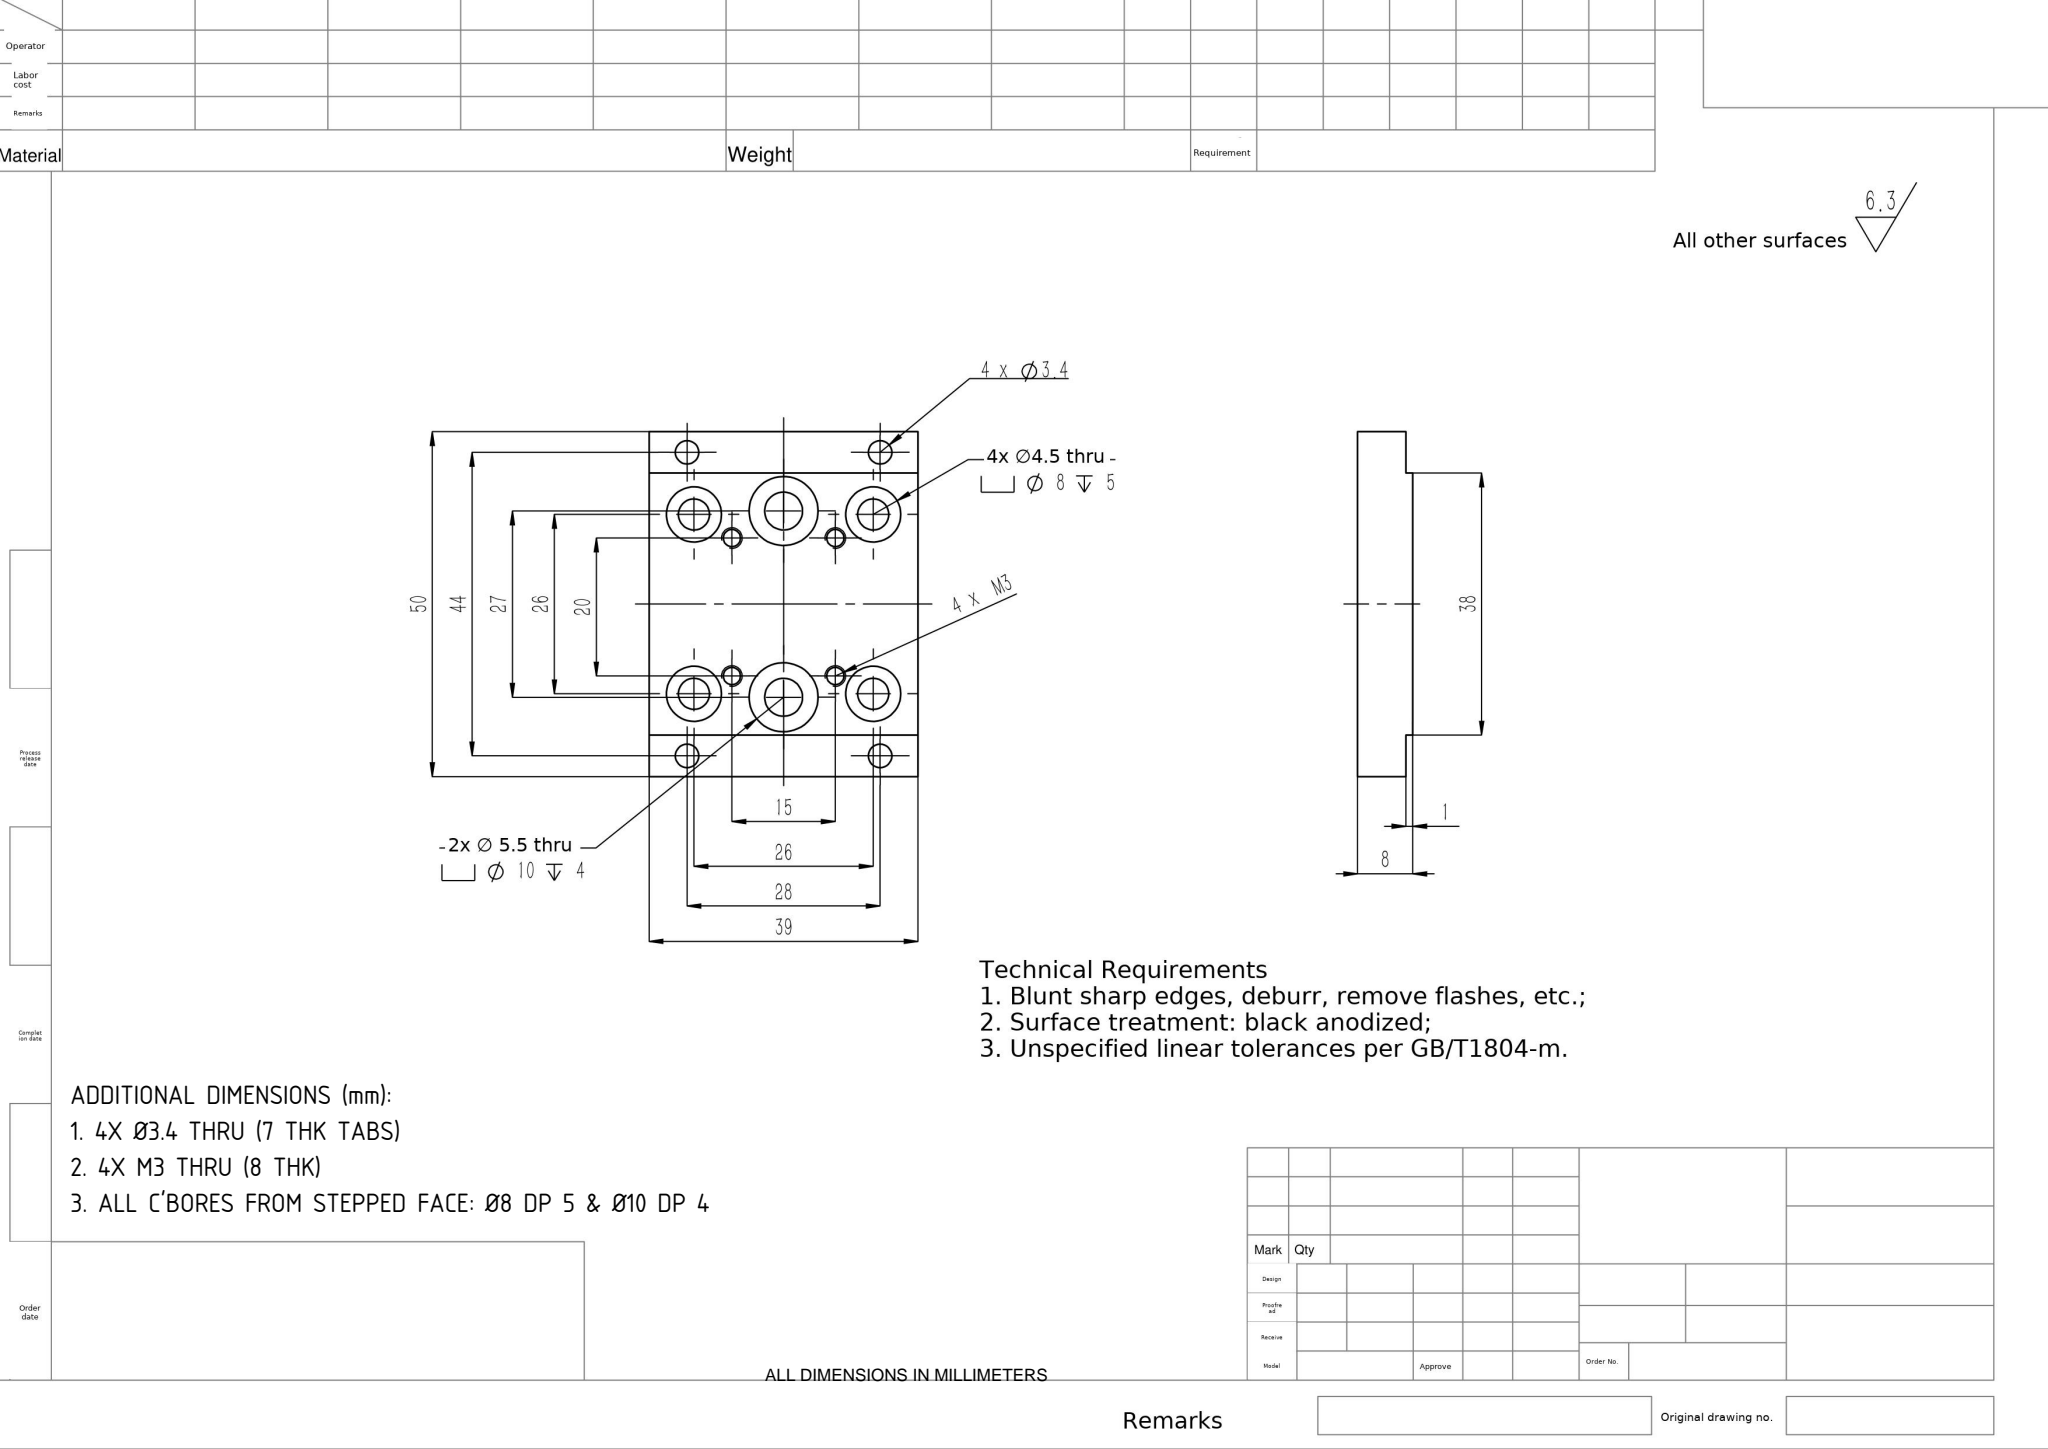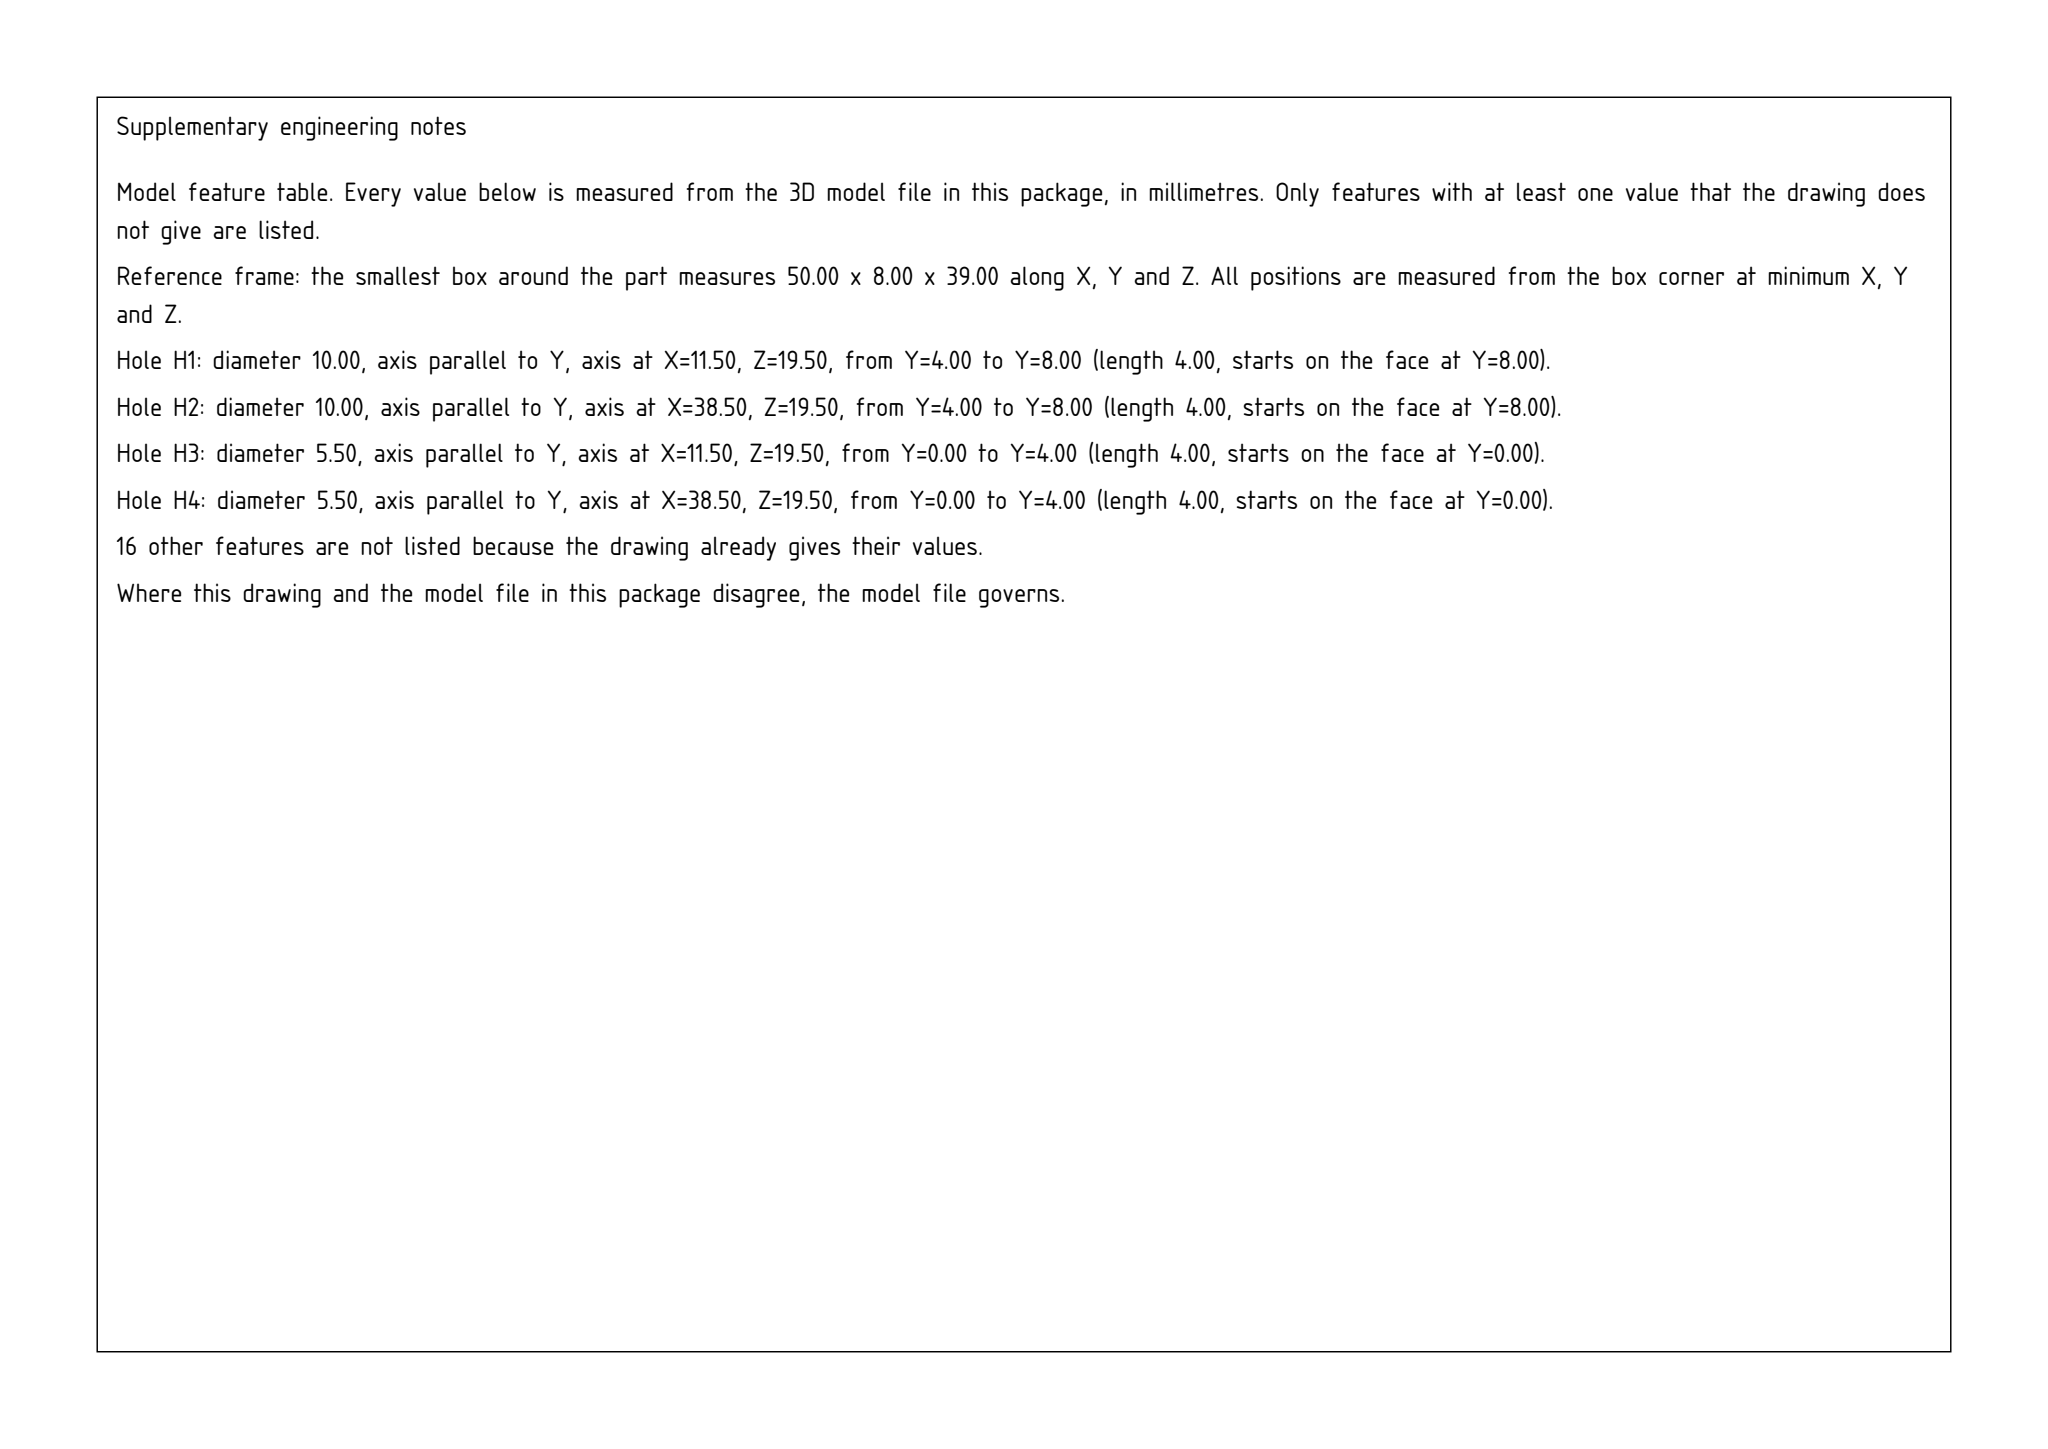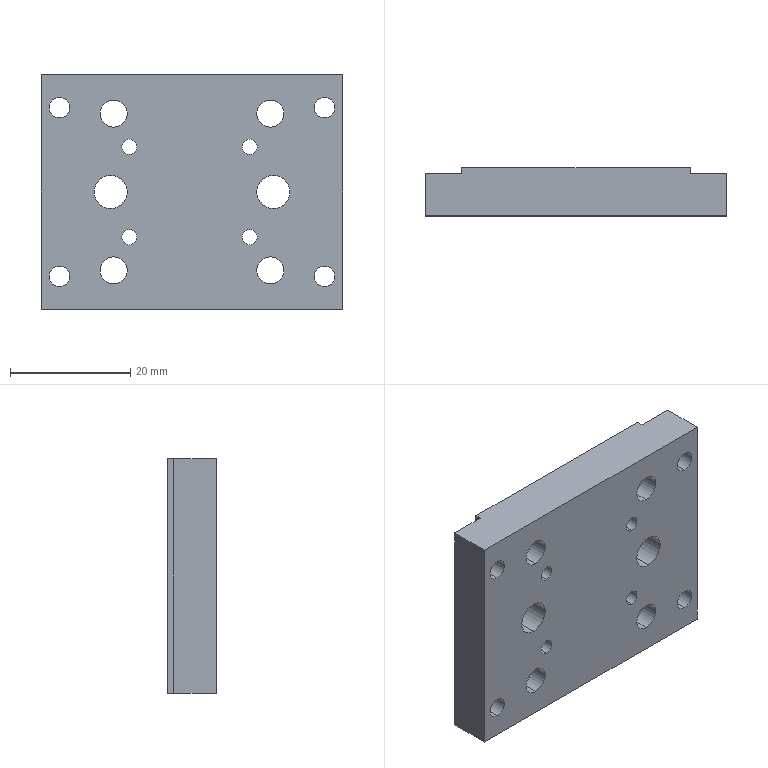Part | SolidWorks | mm | 1 solid | 56 faces | box 50 x 8 x 39 mm | volume 12706 mm3 | cylinder 40 | plane 16 | commonest cylinder face diameters 3.4 x8 2.5 x8 8 x8 4.5 x8 10 x4 5.5 x4
build123d program:
from build123d import *

# Parameters (mm, degrees)
SKETCH1_W                                         = 50
SKETCH1_H                                         = 39
BOSS_EXTRUDE1_DEPTH                               = 8
HOLE_SIZE_ACCORDING_TO_HEXAGON_SOCKET_D           = 4.5
HOLE_SIZE_ACCORDING_TO_HEXAGON_SOCKET_CBORE_D     = 8
HOLE_SIZE_ACCORDING_TO_HEXAGON_SOCKET_CBORE_DEPTH = 5
M3_TAPPED_HOLE1_D                                 = 2.5
SKETCH6_W                                         = 6
SKETCH6_H                                         = 39
CUT_EXTRUDE1_DEPTH                                = 1
M3_CLEARANCE_HOLE_1_D                             = 3.4
HOLE_SIZE_ACCORDING_TO_HEXAGON_SO_2_D             = 5.5
HOLE_SIZE_ACCORDING_TO_HEXAGON_SO_2_CBORE_D       = 10
HOLE_SIZE_ACCORDING_TO_HEXAGON_SO_2_CBORE_DEPTH   = 4


with BuildPart() as part:
    # Sketch1 → Boss-Extrude1 (new body)
    with BuildSketch(Plane(origin=(0, 15.115, 0), x_dir=(1, 0, 0), z_dir=(0, 1, 0))):
        with Locations((-3.099, -279.3)):
            Rectangle(SKETCH1_W, SKETCH1_H)
    extrude(amount=BOSS_EXTRUDE1_DEPTH)

    # Hole Size _ according to_ Hexagon Socket (through all)
    with Locations(Plane(origin=(0, 23.115, 0), x_dir=(1, 0, 0), z_dir=(0, 1, 0))):
        with Locations((-16.099, -266.3), (-16.099, -292.3), (9.901, -292.3), (9.901, -266.3)):
            CounterBoreHole(HOLE_SIZE_ACCORDING_TO_HEXAGON_SOCKET_D / 2, HOLE_SIZE_ACCORDING_TO_HEXAGON_SOCKET_CBORE_D / 2, HOLE_SIZE_ACCORDING_TO_HEXAGON_SOCKET_CBORE_DEPTH)

    # M3 Tapped Hole1 (through all)
    with Locations(Plane(origin=(0, 23.115, 0), x_dir=(1, 0, 0), z_dir=(0, 1, 0))):
        with Locations((-13.52, -271.8), (-13.52, -286.8), (6.48, -286.8), (6.48, -271.8)):
            Hole(M3_TAPPED_HOLE1_D / 2)

    # Sketch6 → Cut-Extrude1 (cut)
    with BuildSketch(Plane(origin=(0, 23.115, 0), x_dir=(1, 0, 0), z_dir=(0, 1, 0))):
        with Locations((18.901, -279.3)):
            Rectangle(SKETCH6_W, SKETCH6_H)
        with Locations((-25.099, -279.3)):
            Rectangle(SKETCH6_W, SKETCH6_H)
    extrude(amount=-CUT_EXTRUDE1_DEPTH, mode=Mode.SUBTRACT)

    # M3 Clearance Hole 1 (through all)
    with Locations(Plane(origin=(0, 15.115, 0), x_dir=(-1, 0, 0), z_dir=(0, -1, 0))):
        with Locations((-18.901, -293.3), (-18.901, -265.3), (25.099, -265.3), (25.099, -293.3)):
            Hole(M3_CLEARANCE_HOLE_1_D / 2)

    # Hole Size _ according to_ Hexagon So 2 (through all)
    with Locations(Plane(origin=(0, 23.115, 0), x_dir=(1, 0, 0), z_dir=(0, 1, 0))):
        with Locations((-16.599, -279.3), (10.401, -279.3)):
            CounterBoreHole(HOLE_SIZE_ACCORDING_TO_HEXAGON_SO_2_D / 2, HOLE_SIZE_ACCORDING_TO_HEXAGON_SO_2_CBORE_D / 2, HOLE_SIZE_ACCORDING_TO_HEXAGON_SO_2_CBORE_DEPTH)


solid = part.part